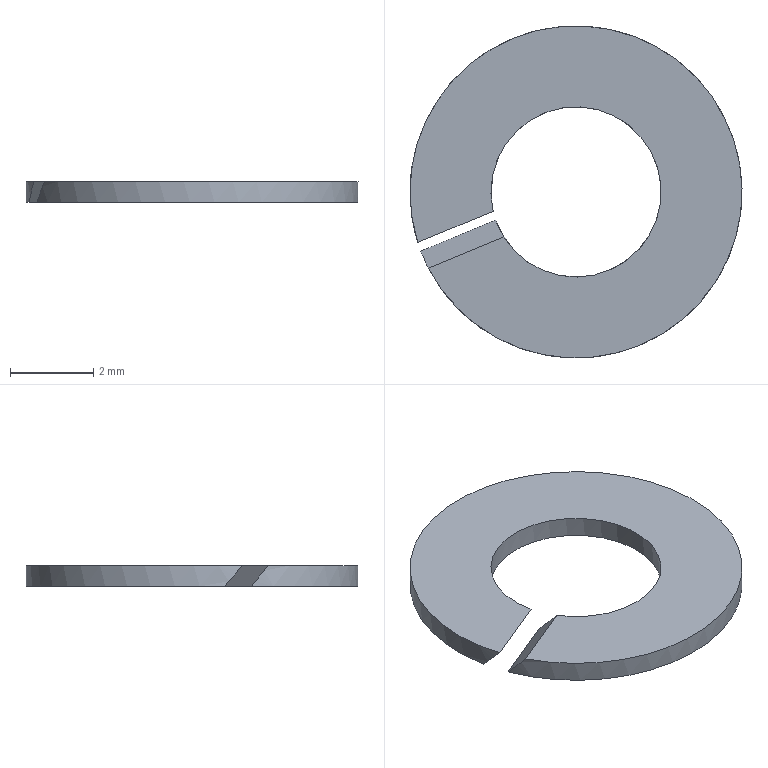Component | NX | SPRING_WASHER_4_3 | 1 solid | 6 faces | box 8 x 8 x 0.5 mm | volume 18 mm3 | plane 4 | cylinder 2 | commonest cylinder face diameters 8 x1 4.1 x1
STEP:
#1=CARTESIAN_POINT('',(0.,0.,0.));
#2=DIRECTION('',(0.,0.,1.));
#3=DIRECTION('',(1.,0.,0.));
#4=AXIS2_PLACEMENT_3D('',#1,#2,#3);
#5=CARTESIAN_POINT('',(-10.811,-1.216,-47.5));
#6=VERTEX_POINT('',#5);
#7=CARTESIAN_POINT('',(-10.924,-0.7757,-48.));
#8=VERTEX_POINT('',#7);
#9=CARTESIAN_POINT('',(-7.,0.,-47.126));
#10=DIRECTION('',(0.2847,-0.6865,-0.6691));
#11=DIRECTION('',(0.2563,-0.6181,0.7431));
#12=AXIS2_PLACEMENT_3D('',#9,#10,#11);
#13=ELLIPSE('',#12,5.978,4.);
#14=CARTESIAN_POINT('',(-7.,0.,-48.));
#15=DIRECTION('',(0.,0.,1.));
#16=DIRECTION('',(0.9237,0.383,0.));
#17=AXIS2_PLACEMENT_3D('',#14,#15,#16);
#18=CYLINDRICAL_SURFACE('',#17,4.);
#19=CARTESIAN_POINT('',(9.341,0.5));
#20=CARTESIAN_POINT('',(9.227,0.));
#21=B_SPLINE_CURVE_WITH_KNOTS('',1,(#19,#20),.UNSPECIFIED.,.F.,.F.,(2,2),(1.655,1.769),.PIECEWISE_BEZIER_KNOTS.);
#22=(GEOMETRIC_REPRESENTATION_CONTEXT(2)PARAMETRIC_REPRESENTATION_CONTEXT()REPRESENTATION_CONTEXT('',''));
#23=DEFINITIONAL_REPRESENTATION('',(#21),#22);
#24=PCURVE('',#18,#23);
#25=CARTESIAN_POINT('',(-17.078,-1.802,-49.565));
#26=DIRECTION('',(-0.2847,0.6865,0.6691));
#27=DIRECTION('',(-0.2563,0.6181,-0.7431));
#28=AXIS2_PLACEMENT_3D('',#25,#26,#27);
#29=PLANE('',#28);
#30=CARTESIAN_POINT('',(-9.259,-10.));
#31=CARTESIAN_POINT('',(-9.259,-3.072));
#32=CARTESIAN_POINT('',(-0.2923,-6.536));
#33=CARTESIAN_POINT('',(8.675,-10.));
#34=CARTESIAN_POINT('',(-0.2923,-13.464));
#35=CARTESIAN_POINT('',(-9.259,-16.928));
#36=CARTESIAN_POINT('',(-9.259,-10.));
#37=(BOUNDED_CURVE()B_SPLINE_CURVE(2,(#30,#31,#32,#33,#34,#35,#36),.UNSPECIFIED.,.T.,.F.)B_SPLINE_CURVE_WITH_KNOTS((1,2,2,2,2,1),(-2.094,0.,2.094,4.189,6.283,8.378),.UNSPECIFIED.)CURVE()GEOMETRIC_REPRESENTATION_ITEM()RATIONAL_B_SPLINE_CURVE((1.,0.5,1.,0.5,1.,0.5,1.))REPRESENTATION_ITEM(''));
#38=(GEOMETRIC_REPRESENTATION_CONTEXT(2)PARAMETRIC_REPRESENTATION_CONTEXT()REPRESENTATION_CONTEXT('',''));
#39=DEFINITIONAL_REPRESENTATION('',(#37),#38);
#40=PCURVE('',#29,#39);
#41=SURFACE_CURVE('',#13,(#24,#40),.PCURVE_S1.);
#42=EDGE_CURVE('',#6,#8,#41,.T.);
#43=ORIENTED_EDGE('',*,*,#42,.F.);
#44=CARTESIAN_POINT('',(-10.553,-1.838,-47.5));
#45=VERTEX_POINT('',#44);
#46=CARTESIAN_POINT('',(-7.,0.,-47.5));
#47=DIRECTION('',(0.,0.,1.));
#48=DIRECTION('',(-0.9237,-0.383,0.));
#49=AXIS2_PLACEMENT_3D('',#46,#47,#48);
#50=CIRCLE('',#49,4.);
#51=CARTESIAN_POINT('',(3.142,0.5));
#52=DIRECTION('',(1.,0.));
#53=VECTOR('',#52,1.);
#54=LINE('',#51,#53);
#55=(GEOMETRIC_REPRESENTATION_CONTEXT(2)PARAMETRIC_REPRESENTATION_CONTEXT()REPRESENTATION_CONTEXT('',''));
#56=DEFINITIONAL_REPRESENTATION('',(#54),#55);
#57=PCURVE('',#18,#56);
#58=CARTESIAN_POINT('',(-7.,0.,-47.5));
#59=DIRECTION('',(0.,0.,1.));
#60=DIRECTION('',(0.9237,0.383,0.));
#61=AXIS2_PLACEMENT_3D('',#58,#59,#60);
#62=PLANE('',#61);
#63=CARTESIAN_POINT('',(0.,0.));
#64=DIRECTION('',(-1.,0.));
#65=AXIS2_PLACEMENT_2D('',#63,#64);
#66=CIRCLE('',#65,4.);
#67=(GEOMETRIC_REPRESENTATION_CONTEXT(2)PARAMETRIC_REPRESENTATION_CONTEXT()REPRESENTATION_CONTEXT('',''));
#68=DEFINITIONAL_REPRESENTATION('',(#66),#67);
#69=PCURVE('',#62,#68);
#70=SURFACE_CURVE('',#50,(#57,#69),.PCURVE_S1.);
#71=EDGE_CURVE('',#45,#6,#70,.T.);
#72=ORIENTED_EDGE('',*,*,#71,.F.);
#73=CARTESIAN_POINT('',(-10.737,-1.426,-48.));
#74=VERTEX_POINT('',#73);
#75=CARTESIAN_POINT('',(-7.,0.,-47.874));
#76=DIRECTION('',(-0.2847,0.6865,0.6691));
#77=DIRECTION('',(0.2563,-0.6181,0.7431));
#78=AXIS2_PLACEMENT_3D('',#75,#76,#77);
#79=ELLIPSE('',#78,5.978,4.);
#80=CARTESIAN_POINT('',(3.113,-0.));
#81=CARTESIAN_POINT('',(3.226,0.5));
#82=B_SPLINE_CURVE_WITH_KNOTS('',1,(#80,#81),.UNSPECIFIED.,.F.,.F.,(2,2),(4.684,4.797),.PIECEWISE_BEZIER_KNOTS.);
#83=(GEOMETRIC_REPRESENTATION_CONTEXT(2)PARAMETRIC_REPRESENTATION_CONTEXT()REPRESENTATION_CONTEXT('',''));
#84=DEFINITIONAL_REPRESENTATION('',(#82),#83);
#85=PCURVE('',#18,#84);
#86=CARTESIAN_POINT('',(-15.396,-5.859,-45.435));
#87=DIRECTION('',(0.2847,-0.6865,-0.6691));
#88=DIRECTION('',(0.2563,-0.6181,0.7431));
#89=AXIS2_PLACEMENT_3D('',#86,#87,#88);
#90=PLANE('',#89);
#91=CARTESIAN_POINT('',(2.697,-10.));
#92=CARTESIAN_POINT('',(2.697,-16.928));
#93=CARTESIAN_POINT('',(-6.27,-13.464));
#94=CARTESIAN_POINT('',(-15.237,-10.));
#95=CARTESIAN_POINT('',(-6.27,-6.536));
#96=CARTESIAN_POINT('',(2.697,-3.072));
#97=CARTESIAN_POINT('',(2.697,-10.));
#98=(BOUNDED_CURVE()B_SPLINE_CURVE(2,(#91,#92,#93,#94,#95,#96,#97),.UNSPECIFIED.,.T.,.F.)B_SPLINE_CURVE_WITH_KNOTS((1,2,2,2,2,1),(-2.094,0.,2.094,4.189,6.283,8.378),.UNSPECIFIED.)CURVE()GEOMETRIC_REPRESENTATION_ITEM()RATIONAL_B_SPLINE_CURVE((1.,0.5,1.,0.5,1.,0.5,1.))REPRESENTATION_ITEM(''));
#99=(GEOMETRIC_REPRESENTATION_CONTEXT(2)PARAMETRIC_REPRESENTATION_CONTEXT()REPRESENTATION_CONTEXT('',''));
#100=DEFINITIONAL_REPRESENTATION('',(#98),#99);
#101=PCURVE('',#90,#100);
#102=SURFACE_CURVE('',#79,(#85,#101),.PCURVE_S1.);
#103=EDGE_CURVE('',#74,#45,#102,.T.);
#104=ORIENTED_EDGE('',*,*,#103,.F.);
#105=CARTESIAN_POINT('',(-7.,0.,-48.));
#106=DIRECTION('',(0.,0.,1.));
#107=DIRECTION('',(-0.9237,-0.383,0.));
#108=AXIS2_PLACEMENT_3D('',#105,#106,#107);
#109=CIRCLE('',#108,4.);
#110=CARTESIAN_POINT('',(-3.142,0.));
#111=DIRECTION('',(1.,0.));
#112=VECTOR('',#111,1.);
#113=LINE('',#110,#112);
#114=(GEOMETRIC_REPRESENTATION_CONTEXT(2)PARAMETRIC_REPRESENTATION_CONTEXT()REPRESENTATION_CONTEXT('',''));
#115=DEFINITIONAL_REPRESENTATION('',(#113),#114);
#116=PCURVE('',#18,#115);
#117=CARTESIAN_POINT('',(-7.,0.,-48.));
#118=DIRECTION('',(0.,0.,1.));
#119=DIRECTION('',(0.9237,0.383,0.));
#120=AXIS2_PLACEMENT_3D('',#117,#118,#119);
#121=PLANE('',#120);
#122=CARTESIAN_POINT('',(0.,0.));
#123=DIRECTION('',(-1.,0.));
#124=AXIS2_PLACEMENT_2D('',#122,#123);
#125=CIRCLE('',#124,4.);
#126=(GEOMETRIC_REPRESENTATION_CONTEXT(2)PARAMETRIC_REPRESENTATION_CONTEXT()REPRESENTATION_CONTEXT('',''));
#127=DEFINITIONAL_REPRESENTATION('',(#125),#126);
#128=PCURVE('',#121,#127);
#129=SURFACE_CURVE('',#109,(#116,#128),.PCURVE_S1.);
#130=EDGE_CURVE('',#74,#8,#129,.T.);
#131=ORIENTED_EDGE('',*,*,#130,.T.);
#132=EDGE_LOOP('',(#43,#72,#104,#131));
#133=FACE_BOUND('',#132,.T.);
#134=ADVANCED_FACE('',(#133),#18,.T.);
#135=CARTESIAN_POINT('',(-8.934,-0.6789,-48.));
#136=VERTEX_POINT('',#135);
#137=CARTESIAN_POINT('',(-8.739,-1.085,-47.5));
#138=VERTEX_POINT('',#137);
#139=CARTESIAN_POINT('',(-7.,0.,-47.874));
#140=DIRECTION('',(-0.2847,0.6865,0.6691));
#141=DIRECTION('',(0.2563,-0.6181,0.7431));
#142=AXIS2_PLACEMENT_3D('',#139,#140,#141);
#143=ELLIPSE('',#142,3.064,2.05);
#144=CARTESIAN_POINT('',(-7.,0.,-48.));
#145=DIRECTION('',(0.,0.,1.));
#146=DIRECTION('',(0.9237,0.383,0.));
#147=AXIS2_PLACEMENT_3D('',#144,#145,#146);
#148=CYLINDRICAL_SURFACE('',#147,2.05);
#149=CARTESIAN_POINT('',(3.086,-0.));
#150=CARTESIAN_POINT('',(3.306,0.5));
#151=B_SPLINE_CURVE_WITH_KNOTS('',1,(#149,#150),.UNSPECIFIED.,.F.,.F.,(2,2),(4.657,4.877),.PIECEWISE_BEZIER_KNOTS.);
#152=(GEOMETRIC_REPRESENTATION_CONTEXT(2)PARAMETRIC_REPRESENTATION_CONTEXT()REPRESENTATION_CONTEXT('',''));
#153=DEFINITIONAL_REPRESENTATION('',(#151),#152);
#154=PCURVE('',#148,#153);
#155=CARTESIAN_POINT('',(-0.2176,-10.));
#156=CARTESIAN_POINT('',(-0.2176,-13.551));
#157=CARTESIAN_POINT('',(-4.813,-11.775));
#158=CARTESIAN_POINT('',(-9.409,-10.));
#159=CARTESIAN_POINT('',(-4.813,-8.225));
#160=CARTESIAN_POINT('',(-0.2176,-6.449));
#161=CARTESIAN_POINT('',(-0.2176,-10.));
#162=(BOUNDED_CURVE()B_SPLINE_CURVE(2,(#155,#156,#157,#158,#159,#160,#161),.UNSPECIFIED.,.T.,.F.)B_SPLINE_CURVE_WITH_KNOTS((1,2,2,2,2,1),(-2.094,0.,2.094,4.189,6.283,8.378),.UNSPECIFIED.)CURVE()GEOMETRIC_REPRESENTATION_ITEM()RATIONAL_B_SPLINE_CURVE((1.,0.5,1.,0.5,1.,0.5,1.))REPRESENTATION_ITEM(''));
#163=(GEOMETRIC_REPRESENTATION_CONTEXT(2)PARAMETRIC_REPRESENTATION_CONTEXT()REPRESENTATION_CONTEXT('',''));
#164=DEFINITIONAL_REPRESENTATION('',(#162),#163);
#165=PCURVE('',#90,#164);
#166=SURFACE_CURVE('',#143,(#154,#165),.PCURVE_S1.);
#167=EDGE_CURVE('',#136,#138,#166,.T.);
#168=ORIENTED_EDGE('',*,*,#167,.F.);
#169=CARTESIAN_POINT('',(-9.05,0.001472,-48.));
#170=VERTEX_POINT('',#169);
#171=CARTESIAN_POINT('',(-7.,0.,-48.));
#172=DIRECTION('',(0.,0.,1.));
#173=DIRECTION('',(-0.9237,-0.383,0.));
#174=AXIS2_PLACEMENT_3D('',#171,#172,#173);
#175=CIRCLE('',#174,2.05);
#176=CARTESIAN_POINT('',(-3.142,0.));
#177=DIRECTION('',(1.,0.));
#178=VECTOR('',#177,1.);
#179=LINE('',#176,#178);
#180=(GEOMETRIC_REPRESENTATION_CONTEXT(2)PARAMETRIC_REPRESENTATION_CONTEXT()REPRESENTATION_CONTEXT('',''));
#181=DEFINITIONAL_REPRESENTATION('',(#179),#180);
#182=PCURVE('',#148,#181);
#183=CARTESIAN_POINT('',(0.,0.));
#184=DIRECTION('',(-1.,0.));
#185=AXIS2_PLACEMENT_2D('',#183,#184);
#186=CIRCLE('',#185,2.05);
#187=(GEOMETRIC_REPRESENTATION_CONTEXT(2)PARAMETRIC_REPRESENTATION_CONTEXT()REPRESENTATION_CONTEXT('',''));
#188=DEFINITIONAL_REPRESENTATION('',(#186),#187);
#189=PCURVE('',#121,#188);
#190=SURFACE_CURVE('',#175,(#182,#189),.PCURVE_S1.);
#191=EDGE_CURVE('',#136,#170,#190,.T.);
#192=ORIENTED_EDGE('',*,*,#191,.T.);
#193=CARTESIAN_POINT('',(-8.997,-0.4639,-47.5));
#194=VERTEX_POINT('',#193);
#195=CARTESIAN_POINT('',(-7.,0.,-47.126));
#196=DIRECTION('',(0.2847,-0.6865,-0.6691));
#197=DIRECTION('',(0.2563,-0.6181,0.7431));
#198=AXIS2_PLACEMENT_3D('',#195,#196,#197);
#199=ELLIPSE('',#198,3.064,2.05);
#200=CARTESIAN_POINT('',(9.26,0.5));
#201=CARTESIAN_POINT('',(9.031,0.));
#202=B_SPLINE_CURVE_WITH_KNOTS('',1,(#200,#201),.UNSPECIFIED.,.F.,.F.,(2,2),(1.736,1.965),.PIECEWISE_BEZIER_KNOTS.);
#203=(GEOMETRIC_REPRESENTATION_CONTEXT(2)PARAMETRIC_REPRESENTATION_CONTEXT()REPRESENTATION_CONTEXT('',''));
#204=DEFINITIONAL_REPRESENTATION('',(#202),#203);
#205=PCURVE('',#148,#204);
#206=CARTESIAN_POINT('',(-6.345,-10.));
#207=CARTESIAN_POINT('',(-6.345,-6.449));
#208=CARTESIAN_POINT('',(-1.749,-8.225));
#209=CARTESIAN_POINT('',(2.846,-10.));
#210=CARTESIAN_POINT('',(-1.749,-11.775));
#211=CARTESIAN_POINT('',(-6.345,-13.551));
#212=CARTESIAN_POINT('',(-6.345,-10.));
#213=(BOUNDED_CURVE()B_SPLINE_CURVE(2,(#206,#207,#208,#209,#210,#211,#212),.UNSPECIFIED.,.T.,.F.)B_SPLINE_CURVE_WITH_KNOTS((1,2,2,2,2,1),(-2.094,0.,2.094,4.189,6.283,8.378),.UNSPECIFIED.)CURVE()GEOMETRIC_REPRESENTATION_ITEM()RATIONAL_B_SPLINE_CURVE((1.,0.5,1.,0.5,1.,0.5,1.))REPRESENTATION_ITEM(''));
#214=(GEOMETRIC_REPRESENTATION_CONTEXT(2)PARAMETRIC_REPRESENTATION_CONTEXT()REPRESENTATION_CONTEXT('',''));
#215=DEFINITIONAL_REPRESENTATION('',(#213),#214);
#216=PCURVE('',#29,#215);
#217=SURFACE_CURVE('',#199,(#205,#216),.PCURVE_S1.);
#218=EDGE_CURVE('',#194,#170,#217,.T.);
#219=ORIENTED_EDGE('',*,*,#218,.F.);
#220=CARTESIAN_POINT('',(-7.,0.,-47.5));
#221=DIRECTION('',(0.,0.,1.));
#222=DIRECTION('',(-0.9237,-0.383,0.));
#223=AXIS2_PLACEMENT_3D('',#220,#221,#222);
#224=CIRCLE('',#223,2.05);
#225=CARTESIAN_POINT('',(3.142,0.5));
#226=DIRECTION('',(1.,0.));
#227=VECTOR('',#226,1.);
#228=LINE('',#225,#227);
#229=(GEOMETRIC_REPRESENTATION_CONTEXT(2)PARAMETRIC_REPRESENTATION_CONTEXT()REPRESENTATION_CONTEXT('',''));
#230=DEFINITIONAL_REPRESENTATION('',(#228),#229);
#231=PCURVE('',#148,#230);
#232=CARTESIAN_POINT('',(0.,0.));
#233=DIRECTION('',(-1.,0.));
#234=AXIS2_PLACEMENT_2D('',#232,#233);
#235=CIRCLE('',#234,2.05);
#236=(GEOMETRIC_REPRESENTATION_CONTEXT(2)PARAMETRIC_REPRESENTATION_CONTEXT()REPRESENTATION_CONTEXT('',''));
#237=DEFINITIONAL_REPRESENTATION('',(#235),#236);
#238=PCURVE('',#62,#237);
#239=SURFACE_CURVE('',#224,(#231,#238),.PCURVE_S1.);
#240=EDGE_CURVE('',#138,#194,#239,.T.);
#241=ORIENTED_EDGE('',*,*,#240,.F.);
#242=EDGE_LOOP('',(#168,#192,#219,#241));
#243=FACE_BOUND('',#242,.F.);
#244=ADVANCED_FACE('',(#243),#148,.F.);
#245=ORIENTED_EDGE('',*,*,#191,.T.);
#246=CARTESIAN_POINT('',(-7.301,0.7266,-48.));
#247=DIRECTION('',(-0.9237,-0.383,0.));
#248=VECTOR('',#247,1.);
#249=LINE('',#246,#248);
#250=CARTESIAN_POINT('',(-0.,0.7866));
#251=DIRECTION('',(-1.,0.));
#252=VECTOR('',#251,1.);
#253=LINE('',#250,#252);
#254=(GEOMETRIC_REPRESENTATION_CONTEXT(2)PARAMETRIC_REPRESENTATION_CONTEXT()REPRESENTATION_CONTEXT('',''));
#255=DEFINITIONAL_REPRESENTATION('',(#253),#254);
#256=PCURVE('',#121,#255);
#257=CARTESIAN_POINT('',(-2.106,-10.));
#258=DIRECTION('',(0.,1.));
#259=VECTOR('',#258,1.);
#260=LINE('',#257,#259);
#261=(GEOMETRIC_REPRESENTATION_CONTEXT(2)PARAMETRIC_REPRESENTATION_CONTEXT()REPRESENTATION_CONTEXT('',''));
#262=DEFINITIONAL_REPRESENTATION('',(#260),#261);
#263=PCURVE('',#29,#262);
#264=SURFACE_CURVE('',#249,(#256,#263),.PCURVE_S1.);
#265=EDGE_CURVE('',#170,#8,#264,.T.);
#266=ORIENTED_EDGE('',*,*,#265,.T.);
#267=ORIENTED_EDGE('',*,*,#130,.F.);
#268=CARTESIAN_POINT('',(-7.044,0.1051,-48.));
#269=DIRECTION('',(0.9237,0.383,0.));
#270=VECTOR('',#269,1.);
#271=LINE('',#268,#270);
#272=CARTESIAN_POINT('',(-0.,0.1138));
#273=DIRECTION('',(1.,0.));
#274=VECTOR('',#273,1.);
#275=LINE('',#272,#274);
#276=(GEOMETRIC_REPRESENTATION_CONTEXT(2)PARAMETRIC_REPRESENTATION_CONTEXT()REPRESENTATION_CONTEXT('',''));
#277=DEFINITIONAL_REPRESENTATION('',(#275),#276);
#278=PCURVE('',#121,#277);
#279=CARTESIAN_POINT('',(-3.451,-10.));
#280=DIRECTION('',(0.,-1.));
#281=VECTOR('',#280,1.);
#282=LINE('',#279,#281);
#283=(GEOMETRIC_REPRESENTATION_CONTEXT(2)PARAMETRIC_REPRESENTATION_CONTEXT()REPRESENTATION_CONTEXT('',''));
#284=DEFINITIONAL_REPRESENTATION('',(#282),#283);
#285=PCURVE('',#90,#284);
#286=SURFACE_CURVE('',#271,(#278,#285),.PCURVE_S1.);
#287=EDGE_CURVE('',#74,#136,#286,.T.);
#288=ORIENTED_EDGE('',*,*,#287,.T.);
#289=EDGE_LOOP('',(#245,#266,#267,#288));
#290=FACE_BOUND('',#289,.T.);
#291=ADVANCED_FACE('',(#290),#121,.F.);
#292=CARTESIAN_POINT('',(-7.129,0.3107,-47.5));
#293=DIRECTION('',(-0.9237,-0.383,0.));
#294=VECTOR('',#293,1.);
#295=LINE('',#292,#294);
#296=CARTESIAN_POINT('',(-0.,0.3364));
#297=DIRECTION('',(-1.,0.));
#298=VECTOR('',#297,1.);
#299=LINE('',#296,#298);
#300=(GEOMETRIC_REPRESENTATION_CONTEXT(2)PARAMETRIC_REPRESENTATION_CONTEXT()REPRESENTATION_CONTEXT('',''));
#301=DEFINITIONAL_REPRESENTATION('',(#299),#300);
#302=PCURVE('',#62,#301);
#303=CARTESIAN_POINT('',(-2.779,-10.));
#304=DIRECTION('',(0.,1.));
#305=VECTOR('',#304,1.);
#306=LINE('',#303,#305);
#307=(GEOMETRIC_REPRESENTATION_CONTEXT(2)PARAMETRIC_REPRESENTATION_CONTEXT()REPRESENTATION_CONTEXT('',''));
#308=DEFINITIONAL_REPRESENTATION('',(#306),#307);
#309=PCURVE('',#29,#308);
#310=SURFACE_CURVE('',#295,(#302,#309),.PCURVE_S1.);
#311=EDGE_CURVE('',#194,#6,#310,.T.);
#312=ORIENTED_EDGE('',*,*,#311,.F.);
#313=ORIENTED_EDGE('',*,*,#240,.F.);
#314=CARTESIAN_POINT('',(-6.871,-0.3107,-47.5));
#315=DIRECTION('',(0.9237,0.383,0.));
#316=VECTOR('',#315,1.);
#317=LINE('',#314,#316);
#318=CARTESIAN_POINT('',(-0.,-0.3364));
#319=DIRECTION('',(1.,0.));
#320=VECTOR('',#319,1.);
#321=LINE('',#318,#320);
#322=(GEOMETRIC_REPRESENTATION_CONTEXT(2)PARAMETRIC_REPRESENTATION_CONTEXT()REPRESENTATION_CONTEXT('',''));
#323=DEFINITIONAL_REPRESENTATION('',(#321),#322);
#324=PCURVE('',#62,#323);
#325=CARTESIAN_POINT('',(-2.779,-10.));
#326=DIRECTION('',(0.,-1.));
#327=VECTOR('',#326,1.);
#328=LINE('',#325,#327);
#329=(GEOMETRIC_REPRESENTATION_CONTEXT(2)PARAMETRIC_REPRESENTATION_CONTEXT()REPRESENTATION_CONTEXT('',''));
#330=DEFINITIONAL_REPRESENTATION('',(#328),#329);
#331=PCURVE('',#90,#330);
#332=SURFACE_CURVE('',#317,(#324,#331),.PCURVE_S1.);
#333=EDGE_CURVE('',#45,#138,#332,.T.);
#334=ORIENTED_EDGE('',*,*,#333,.F.);
#335=ORIENTED_EDGE('',*,*,#71,.T.);
#336=EDGE_LOOP('',(#312,#313,#334,#335));
#337=FACE_BOUND('',#336,.T.);
#338=ADVANCED_FACE('',(#337),#62,.T.);
#339=ORIENTED_EDGE('',*,*,#103,.T.);
#340=ORIENTED_EDGE('',*,*,#333,.T.);
#341=ORIENTED_EDGE('',*,*,#167,.F.);
#342=ORIENTED_EDGE('',*,*,#287,.F.);
#343=EDGE_LOOP('',(#339,#340,#341,#342));
#344=FACE_BOUND('',#343,.T.);
#345=ADVANCED_FACE('',(#344),#90,.F.);
#346=ORIENTED_EDGE('',*,*,#218,.F.);
#347=ORIENTED_EDGE('',*,*,#311,.T.);
#348=ORIENTED_EDGE('',*,*,#42,.T.);
#349=ORIENTED_EDGE('',*,*,#265,.F.);
#350=EDGE_LOOP('',(#346,#347,#348,#349));
#351=FACE_BOUND('',#350,.T.);
#352=ADVANCED_FACE('',(#351),#29,.F.);
#353=CLOSED_SHELL('',(#134,#244,#291,#338,#345,#352));
#354=MANIFOLD_SOLID_BREP('',#353);
#355=(LENGTH_UNIT()NAMED_UNIT(*)SI_UNIT(.MILLI.,.METRE.));
#356=UNCERTAINTY_MEASURE_WITH_UNIT(LENGTH_MEASURE(0.001),#355,'','');
#357=(NAMED_UNIT(*)PLANE_ANGLE_UNIT()SI_UNIT($,.RADIAN.));
#358=(NAMED_UNIT(*)SI_UNIT($,.STERADIAN.)SOLID_ANGLE_UNIT());
#359=(GEOMETRIC_REPRESENTATION_CONTEXT(3)GLOBAL_UNCERTAINTY_ASSIGNED_CONTEXT((#356))GLOBAL_UNIT_ASSIGNED_CONTEXT((#355,#357,#358))REPRESENTATION_CONTEXT('',''));
#360=ADVANCED_BREP_SHAPE_REPRESENTATION('',(#4,#354),#359);